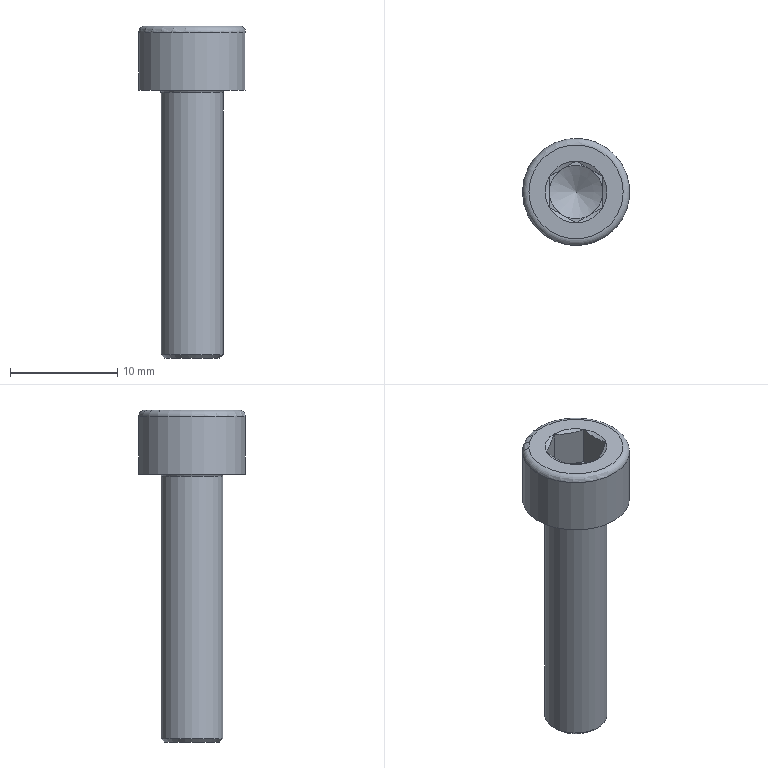Component | NX | GB-T70_1-2000_M6X25_3 | 1 solid | 27 faces | volume 1038 mm3 | plane 15 | cone 8 | cylinder 2 | torus 2 | commonest cylinder face diameters 5.795 x1 10 x1